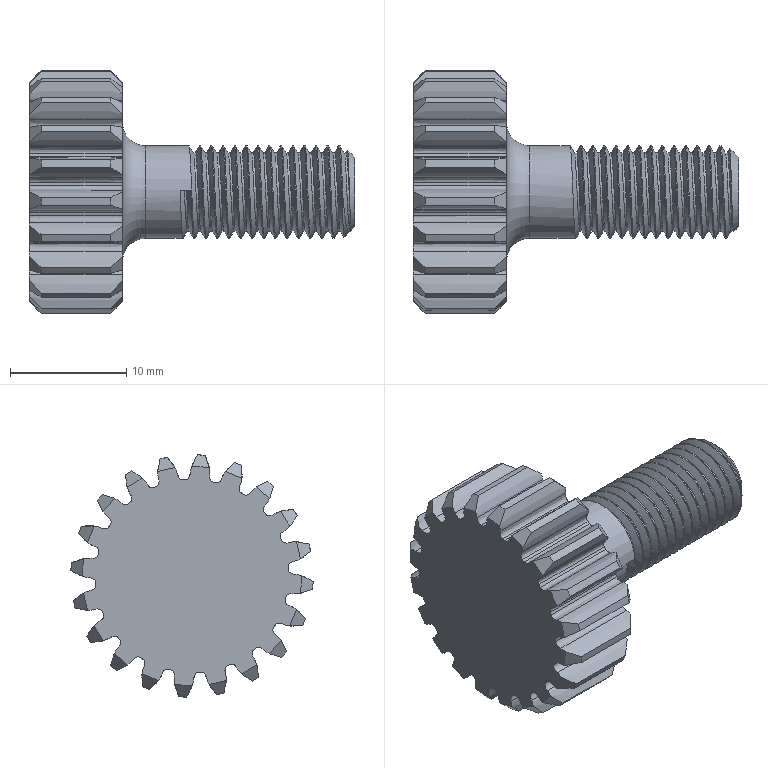Component | NX | LOCKING_SCREW | 1 solid | 185 faces | volume 3102 mm3 | other 100 | spline 42 | cylinder 36 | plane 4 | cone 2 | torus 1 | commonest cylinder face diameters 16.625 x20 8 x15 6.75 x1